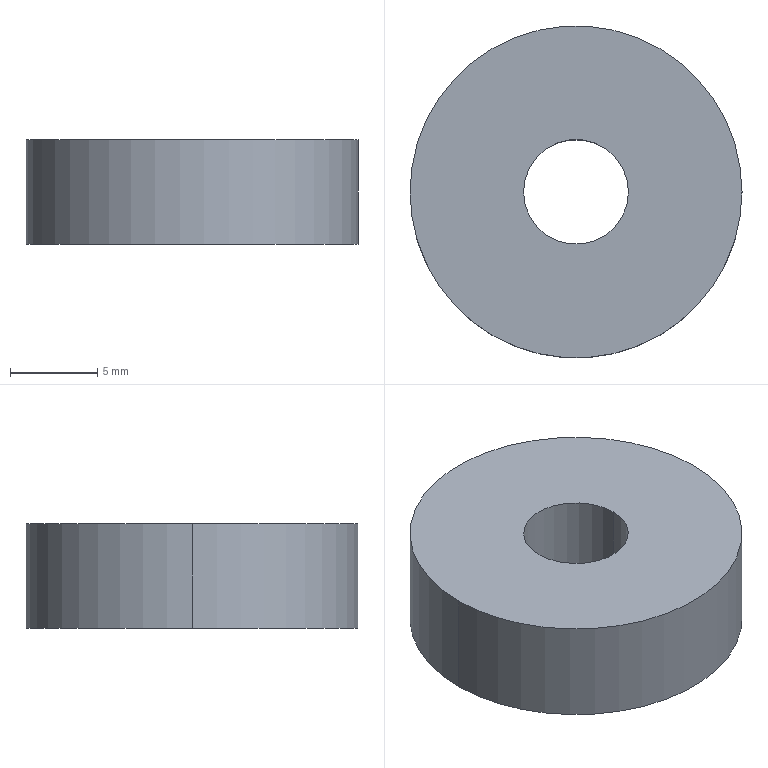Component | SolidWorks | Bearing626z-1 | 1 solid | 6 faces | box 19 x 19 x 6 mm | volume 1532 mm3 | cylinder 4 | plane 2 | commonest cylinder face diameters 6 x2 19 x2
build123d program:
from build123d import *

# Parameters (mm, degrees)
SKETCH1_R      = 9.5
SKETCH1_R_2    = 3
EXTRUDE1_DEPTH = 6


with BuildPart() as part:
    # Sketch1 → Extrude1 (new body)
    with BuildSketch(Plane.XY):
        Circle(SKETCH1_R)
        Circle(SKETCH1_R_2, mode=Mode.SUBTRACT)
    extrude(amount=EXTRUDE1_DEPTH)


solid = part.part

# Placed as in the assembly
solid = solid.moved(Location((-108.621, -15.488, -4.189), (0, 0, 0)))
STEP:
#1=COLOUR_RGB('',0.7922,0.8196,0.9333);
#2=FILL_AREA_STYLE_COLOUR('',#1);
#3=FILL_AREA_STYLE('',(#2));
#4=SURFACE_STYLE_FILL_AREA(#3);
#5=SURFACE_SIDE_STYLE('',(#4));
#6=SURFACE_STYLE_USAGE(.BOTH.,#5);
#7=PRESENTATION_STYLE_ASSIGNMENT((#6));
#8=CARTESIAN_POINT('',(-4.158,-0.6098,0.07129));
#9=VERTEX_POINT('',#8);
#10=CARTESIAN_POINT('',(-4.395,-0.6098,0.07129));
#11=VERTEX_POINT('',#10);
#12=CARTESIAN_POINT('',(-4.276,-0.6098,0.07129));
#13=DIRECTION('',(0.,0.,1.));
#14=DIRECTION('',(-1.,0.,0.));
#15=AXIS2_PLACEMENT_3D('',#12,#13,#14);
#16=CIRCLE('',#15,0.1181);
#17=EDGE_CURVE('',#9,#11,#16,.T.);
#18=ORIENTED_EDGE('',*,*,#17,.T.);
#19=CARTESIAN_POINT('',(-4.395,-0.6098,-0.1649));
#20=VERTEX_POINT('',#19);
#21=CARTESIAN_POINT('',(-4.395,-0.6098,0.07129));
#22=DIRECTION('',(0.,0.,-1.));
#23=VECTOR('',#22,39.37);
#24=LINE('',#21,#23);
#25=EDGE_CURVE('',#11,#20,#24,.T.);
#26=ORIENTED_EDGE('',*,*,#25,.T.);
#27=CARTESIAN_POINT('',(-4.158,-0.6098,-0.1649));
#28=VERTEX_POINT('',#27);
#29=CARTESIAN_POINT('',(-4.276,-0.6098,-0.1649));
#30=DIRECTION('',(0.,0.,1.));
#31=DIRECTION('',(-1.,0.,0.));
#32=AXIS2_PLACEMENT_3D('',#29,#30,#31);
#33=CIRCLE('',#32,0.1181);
#34=EDGE_CURVE('',#28,#20,#33,.T.);
#35=ORIENTED_EDGE('',*,*,#34,.F.);
#36=CARTESIAN_POINT('',(-4.158,-0.6098,0.07129));
#37=DIRECTION('',(0.,0.,-1.));
#38=VECTOR('',#37,39.37);
#39=LINE('',#36,#38);
#40=EDGE_CURVE('',#9,#28,#39,.T.);
#41=ORIENTED_EDGE('',*,*,#40,.F.);
#42=EDGE_LOOP('',(#18,#26,#35,#41));
#43=FACE_OUTER_BOUND('',#42,.T.);
#44=CARTESIAN_POINT('',(-4.276,-0.6098,0.07129));
#45=DIRECTION('',(0.,0.,-1.));
#46=DIRECTION('',(1.,0.,0.));
#47=AXIS2_PLACEMENT_3D('',#44,#45,#46);
#48=CYLINDRICAL_SURFACE('',#47,0.1181);
#49=ADVANCED_FACE('',(#43),#48,.F.);
#50=CARTESIAN_POINT('',(-4.65,-0.6098,0.07129));
#51=VERTEX_POINT('',#50);
#52=CARTESIAN_POINT('',(-3.902,-0.6098,0.07129));
#53=VERTEX_POINT('',#52);
#54=CARTESIAN_POINT('',(-4.276,-0.6098,0.07129));
#55=DIRECTION('',(0.,0.,1.));
#56=DIRECTION('',(-1.,-0.,0.));
#57=AXIS2_PLACEMENT_3D('',#54,#55,#56);
#58=CIRCLE('',#57,0.374);
#59=EDGE_CURVE('',#51,#53,#58,.T.);
#60=ORIENTED_EDGE('',*,*,#59,.F.);
#61=CARTESIAN_POINT('',(-4.65,-0.6098,-0.1649));
#62=VERTEX_POINT('',#61);
#63=CARTESIAN_POINT('',(-4.65,-0.6098,0.07129));
#64=DIRECTION('',(0.,0.,-1.));
#65=VECTOR('',#64,39.37);
#66=LINE('',#63,#65);
#67=EDGE_CURVE('',#51,#62,#66,.T.);
#68=ORIENTED_EDGE('',*,*,#67,.T.);
#69=CARTESIAN_POINT('',(-3.902,-0.6098,-0.1649));
#70=VERTEX_POINT('',#69);
#71=CARTESIAN_POINT('',(-4.276,-0.6098,-0.1649));
#72=DIRECTION('',(0.,0.,1.));
#73=DIRECTION('',(-1.,-0.,0.));
#74=AXIS2_PLACEMENT_3D('',#71,#72,#73);
#75=CIRCLE('',#74,0.374);
#76=EDGE_CURVE('',#62,#70,#75,.T.);
#77=ORIENTED_EDGE('',*,*,#76,.T.);
#78=CARTESIAN_POINT('',(-3.902,-0.6098,0.07129));
#79=DIRECTION('',(0.,0.,-1.));
#80=VECTOR('',#79,39.37);
#81=LINE('',#78,#80);
#82=EDGE_CURVE('',#53,#70,#81,.T.);
#83=ORIENTED_EDGE('',*,*,#82,.F.);
#84=EDGE_LOOP('',(#60,#68,#77,#83));
#85=FACE_OUTER_BOUND('',#84,.T.);
#86=CARTESIAN_POINT('',(-4.276,-0.6098,0.07129));
#87=DIRECTION('',(0.,0.,-1.));
#88=DIRECTION('',(1.,0.,0.));
#89=AXIS2_PLACEMENT_3D('',#86,#87,#88);
#90=CYLINDRICAL_SURFACE('',#89,0.374);
#91=ADVANCED_FACE('',(#85),#90,.T.);
#92=CARTESIAN_POINT('',(-4.276,-0.6098,0.07129));
#93=DIRECTION('',(0.,0.,1.));
#94=DIRECTION('',(-1.,-0.,0.));
#95=AXIS2_PLACEMENT_3D('',#92,#93,#94);
#96=CIRCLE('',#95,0.374);
#97=EDGE_CURVE('',#53,#51,#96,.T.);
#98=ORIENTED_EDGE('',*,*,#97,.T.);
#99=ORIENTED_EDGE('',*,*,#59,.T.);
#100=EDGE_LOOP('',(#98,#99));
#101=FACE_OUTER_BOUND('',#100,.T.);
#102=ORIENTED_EDGE('',*,*,#17,.F.);
#103=CARTESIAN_POINT('',(-4.276,-0.6098,0.07129));
#104=DIRECTION('',(0.,0.,1.));
#105=DIRECTION('',(-1.,0.,0.));
#106=AXIS2_PLACEMENT_3D('',#103,#104,#105);
#107=CIRCLE('',#106,0.1181);
#108=EDGE_CURVE('',#11,#9,#107,.T.);
#109=ORIENTED_EDGE('',*,*,#108,.F.);
#110=EDGE_LOOP('',(#102,#109));
#111=FACE_BOUND('',#110,.T.);
#112=CARTESIAN_POINT('',(-4.276,-0.6098,0.07129));
#113=DIRECTION('',(0.,0.,1.));
#114=DIRECTION('',(-1.,-0.,0.));
#115=AXIS2_PLACEMENT_3D('',#112,#113,#114);
#116=PLANE('',#115);
#117=ADVANCED_FACE('',(#101,#111),#116,.T.);
#118=CARTESIAN_POINT('',(-4.276,-0.6098,-0.1649));
#119=DIRECTION('',(0.,0.,1.));
#120=DIRECTION('',(-1.,-0.,0.));
#121=AXIS2_PLACEMENT_3D('',#118,#119,#120);
#122=CIRCLE('',#121,0.374);
#123=EDGE_CURVE('',#70,#62,#122,.T.);
#124=ORIENTED_EDGE('',*,*,#123,.F.);
#125=ORIENTED_EDGE('',*,*,#76,.F.);
#126=EDGE_LOOP('',(#124,#125));
#127=FACE_OUTER_BOUND('',#126,.T.);
#128=ORIENTED_EDGE('',*,*,#34,.T.);
#129=CARTESIAN_POINT('',(-4.276,-0.6098,-0.1649));
#130=DIRECTION('',(0.,0.,1.));
#131=DIRECTION('',(-1.,0.,0.));
#132=AXIS2_PLACEMENT_3D('',#129,#130,#131);
#133=CIRCLE('',#132,0.1181);
#134=EDGE_CURVE('',#20,#28,#133,.T.);
#135=ORIENTED_EDGE('',*,*,#134,.T.);
#136=EDGE_LOOP('',(#128,#135));
#137=FACE_BOUND('',#136,.T.);
#138=CARTESIAN_POINT('',(-4.276,-0.6098,-0.1649));
#139=DIRECTION('',(0.,0.,1.));
#140=DIRECTION('',(-1.,-0.,0.));
#141=AXIS2_PLACEMENT_3D('',#138,#139,#140);
#142=PLANE('',#141);
#143=ADVANCED_FACE('',(#127,#137),#142,.F.);
#144=ORIENTED_EDGE('',*,*,#67,.F.);
#145=ORIENTED_EDGE('',*,*,#97,.F.);
#146=ORIENTED_EDGE('',*,*,#82,.T.);
#147=ORIENTED_EDGE('',*,*,#123,.T.);
#148=EDGE_LOOP('',(#144,#145,#146,#147));
#149=FACE_OUTER_BOUND('',#148,.T.);
#150=CARTESIAN_POINT('',(-4.276,-0.6098,0.07129));
#151=DIRECTION('',(0.,0.,-1.));
#152=DIRECTION('',(1.,0.,0.));
#153=AXIS2_PLACEMENT_3D('',#150,#151,#152);
#154=CYLINDRICAL_SURFACE('',#153,0.374);
#155=ADVANCED_FACE('',(#149),#154,.T.);
#156=ORIENTED_EDGE('',*,*,#25,.F.);
#157=ORIENTED_EDGE('',*,*,#108,.T.);
#158=ORIENTED_EDGE('',*,*,#40,.T.);
#159=ORIENTED_EDGE('',*,*,#134,.F.);
#160=EDGE_LOOP('',(#156,#157,#158,#159));
#161=FACE_OUTER_BOUND('',#160,.T.);
#162=CARTESIAN_POINT('',(-4.276,-0.6098,0.07129));
#163=DIRECTION('',(0.,0.,-1.));
#164=DIRECTION('',(1.,0.,0.));
#165=AXIS2_PLACEMENT_3D('',#162,#163,#164);
#166=CYLINDRICAL_SURFACE('',#165,0.1181);
#167=ADVANCED_FACE('',(#161),#166,.F.);
#168=CLOSED_SHELL('',(#49,#91,#117,#143,#155,#167));
#169=MANIFOLD_SOLID_BREP('',#168);
#170=STYLED_ITEM('',(#7),#169);
#171=(LENGTH_UNIT()NAMED_UNIT(*)SI_UNIT($,.METRE.));
#172=LENGTH_MEASURE_WITH_UNIT(LENGTH_MEASURE(0.0254),#171);
#173=DIMENSIONAL_EXPONENTS(1.,0.,0.,0.,0.,0.,0.);
#174=(CONVERSION_BASED_UNIT('',#172)LENGTH_UNIT()NAMED_UNIT(#173));
#175=UNCERTAINTY_MEASURE_WITH_UNIT(LENGTH_MEASURE(0.00001),#174,'','');
#176=(NAMED_UNIT(*)PLANE_ANGLE_UNIT()SI_UNIT($,.RADIAN.));
#177=(NAMED_UNIT(*)SI_UNIT($,.STERADIAN.)SOLID_ANGLE_UNIT());
#178=(GEOMETRIC_REPRESENTATION_CONTEXT(3)GLOBAL_UNCERTAINTY_ASSIGNED_CONTEXT((#175))GLOBAL_UNIT_ASSIGNED_CONTEXT((#174,#176,#177))REPRESENTATION_CONTEXT('',''));
#179=MECHANICAL_DESIGN_GEOMETRIC_PRESENTATION_REPRESENTATION('',(#170),#178);
#180=PRESENTATION_LAYER_ASSIGNMENT('','',(#170));
#181=CARTESIAN_POINT('',(0.,0.,0.));
#182=DIRECTION('',(0.,0.,1.));
#183=DIRECTION('',(1.,0.,0.));
#184=AXIS2_PLACEMENT_3D('',#181,#182,#183);
#185=(LENGTH_UNIT()NAMED_UNIT(*)SI_UNIT($,.METRE.));
#186=LENGTH_MEASURE_WITH_UNIT(LENGTH_MEASURE(0.0254),#185);
#187=DIMENSIONAL_EXPONENTS(1.,0.,0.,0.,0.,0.,0.);
#188=(CONVERSION_BASED_UNIT('',#186)LENGTH_UNIT()NAMED_UNIT(#187));
#189=UNCERTAINTY_MEASURE_WITH_UNIT(LENGTH_MEASURE(0.00001),#188,'','');
#190=(NAMED_UNIT(*)PLANE_ANGLE_UNIT()SI_UNIT($,.RADIAN.));
#191=(NAMED_UNIT(*)SI_UNIT($,.STERADIAN.)SOLID_ANGLE_UNIT());
#192=(GEOMETRIC_REPRESENTATION_CONTEXT(3)GLOBAL_UNCERTAINTY_ASSIGNED_CONTEXT((#189))GLOBAL_UNIT_ASSIGNED_CONTEXT((#188,#190,#191))REPRESENTATION_CONTEXT('',''));
#193=ADVANCED_BREP_SHAPE_REPRESENTATION('',(#169,#184),#192);